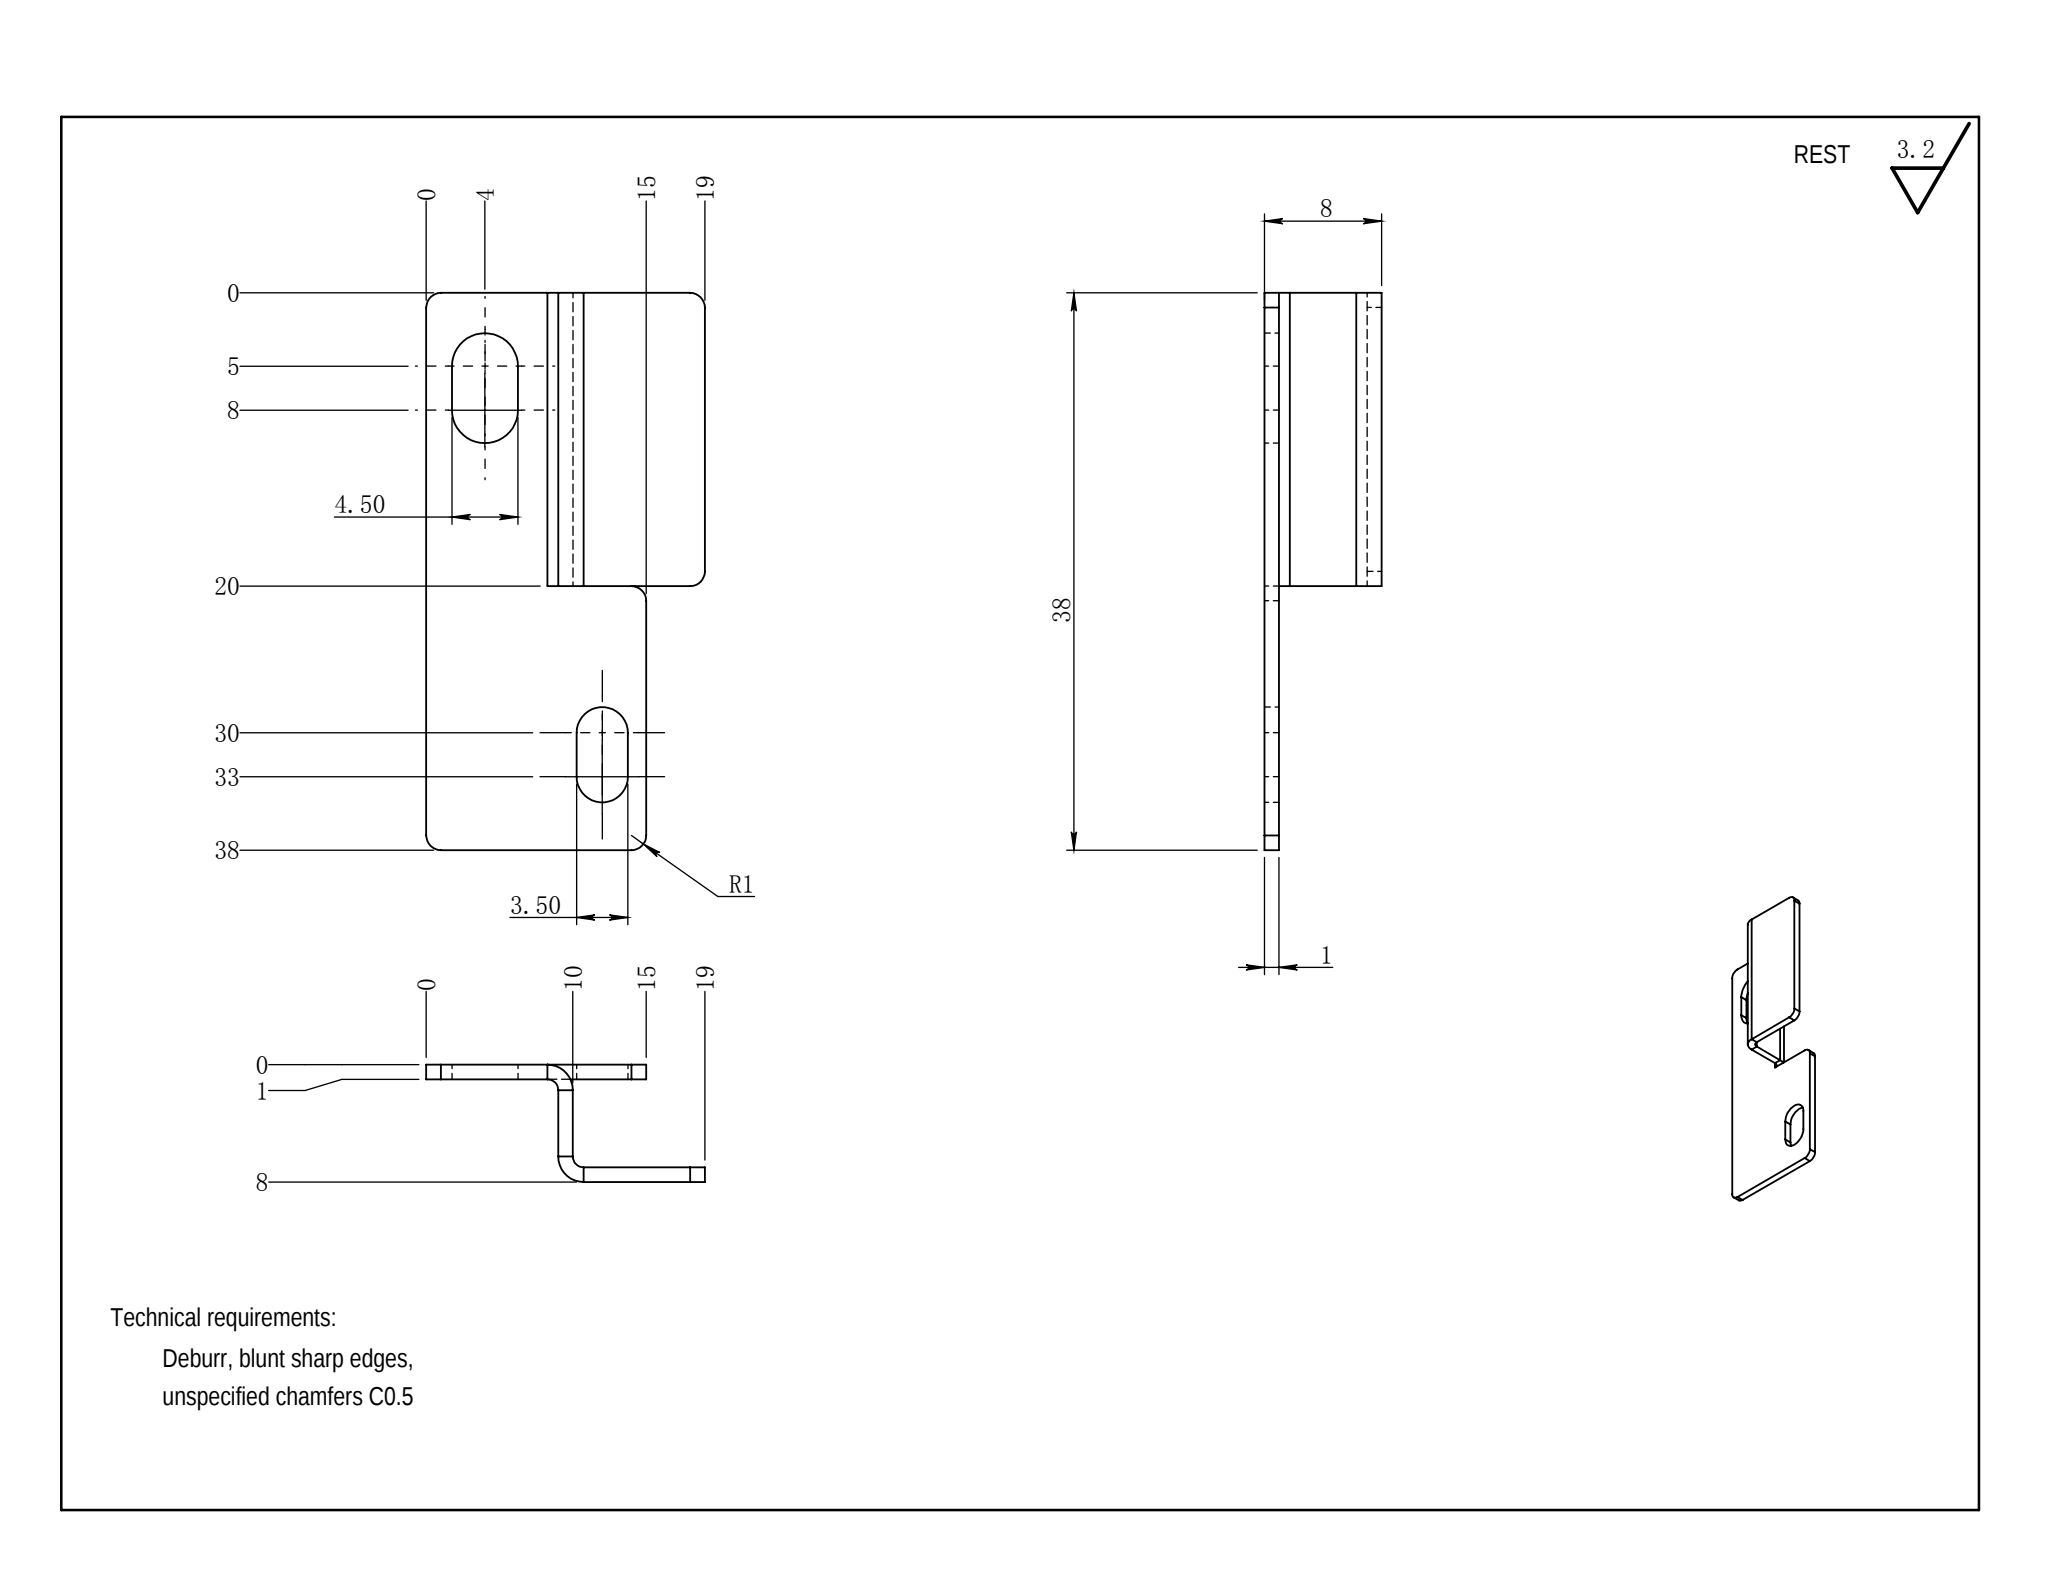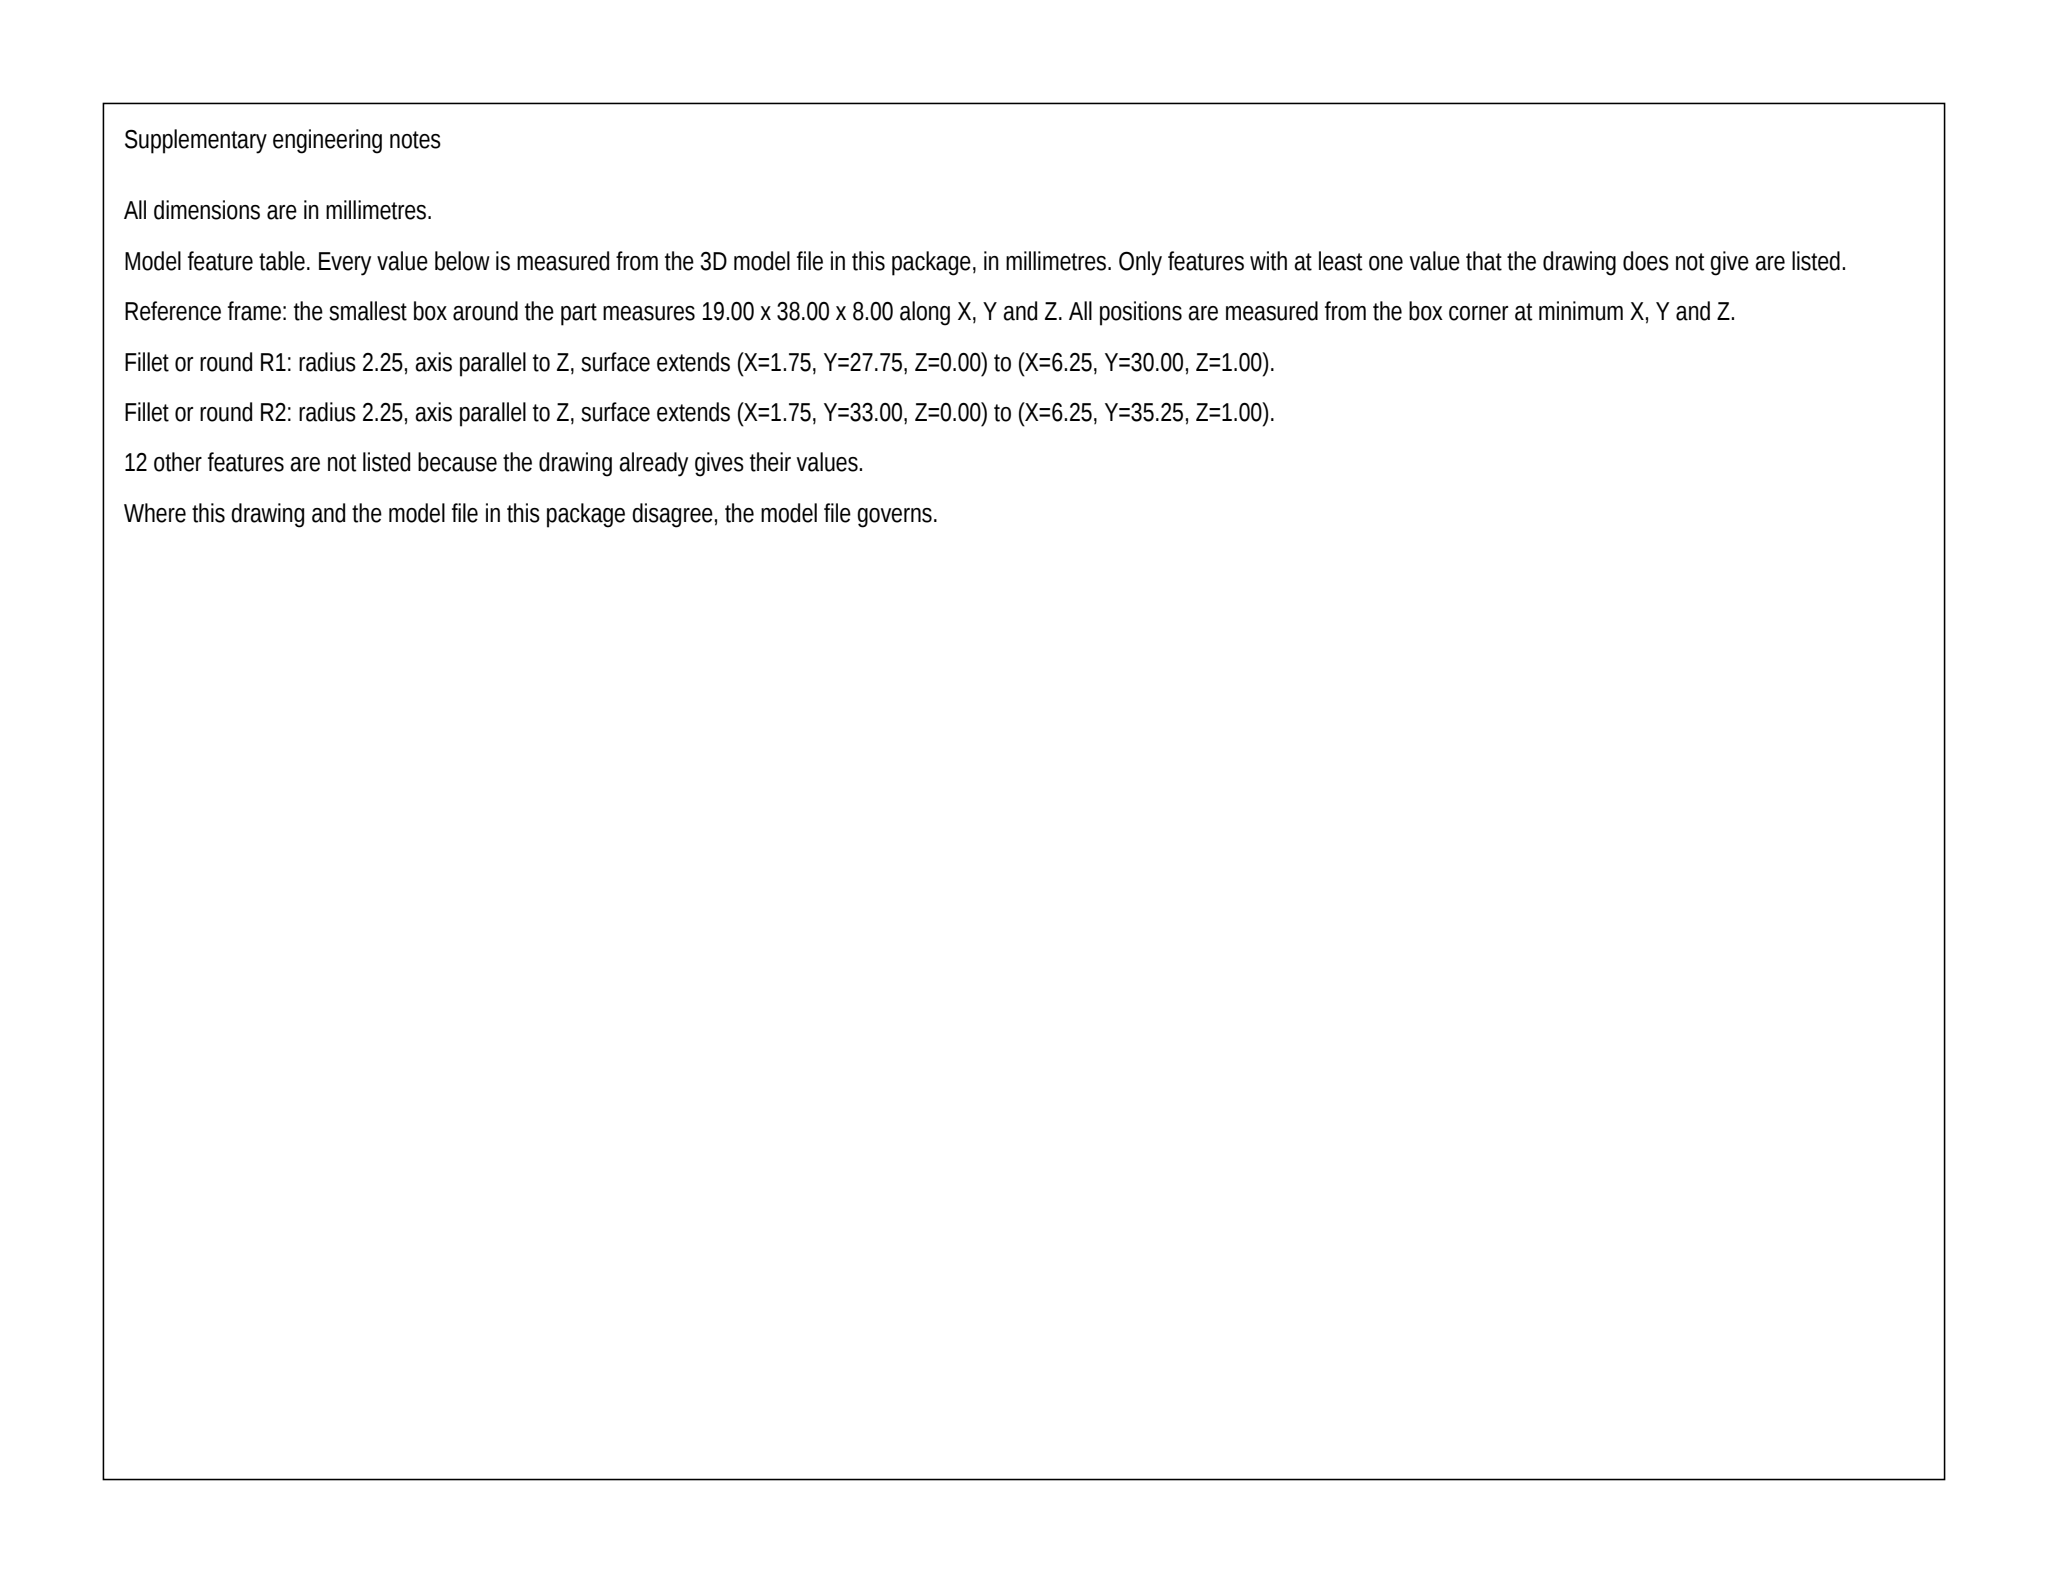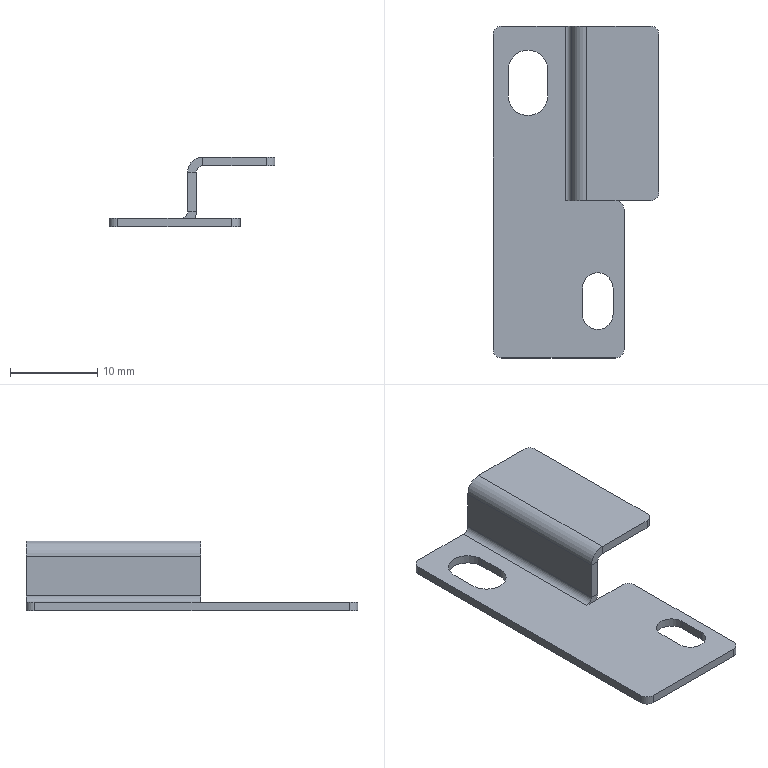Part | SolidWorks | mm | 1 solid | 38 faces | box 19 x 38 x 8 mm | volume 718 mm3 | plane 24 | cylinder 14 | commonest cylinder face diameters 2 x6 3.473 x2 1.473 x2 4.5 x2 3.5 x2